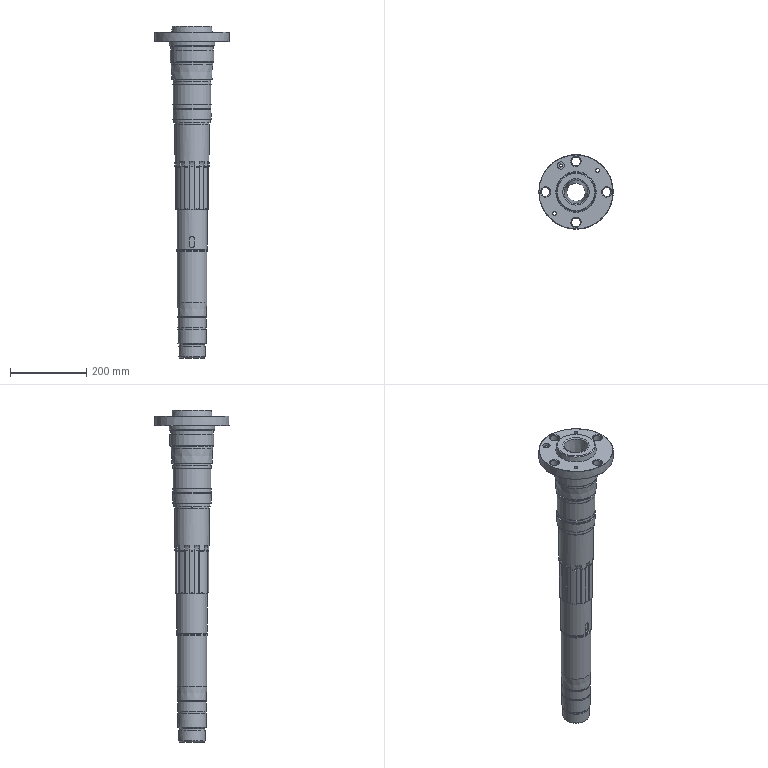Component | NX | CA6140-ZHUZHOU | 1 solid | 197 faces | volume 4103501 mm3 | plane 69 | cylinder 67 | cone 35 | torus 26 | commonest cylinder face diameters 81.6 x10 86 x10 89 x10 23 x4 100 x3 80 x2 97 x2 12 x2